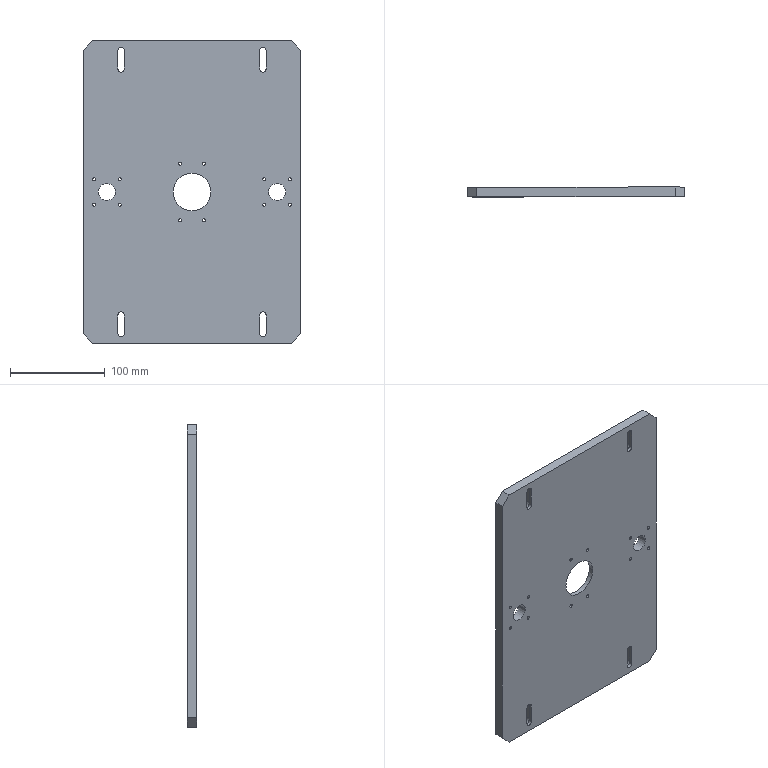Component | SolidWorks | UpperAndLowerCylinderMountingPlate-1 | 1 solid | 85 faces | box 230 x 10.04 x 320 mm | volume 691383 mm3 | cylinder 50 | plane 35 | commonest cylinder face diameters 3.3 x24 11 x8 6.6 x8 18 x4 8 x4 40 x2
build123d program:
from build123d import *

# Parameters (mm, degrees)
SKETCH1_W                                       = 230
SKETCH1_H                                       = 320
BOSS_EXTRUDE1_DEPTH                             = 10
SKETCH2_R                                       = 9
CUT_EXTRUDE1_DEPTH                              = 10
SKETCH3_R                                       = 20
CUT_EXTRUDE2_DEPTH                              = 10
CHAMFER1_SIZE                                   = 10
M4_TAPPED_HOLE1_D                               = 3.3
SKETCH6_W                                       = 50
SKETCH6_H                                       = 80
CUT_EXTRUDE3_DEPTH                              = 5
FILLET1_R                                       = 4
M4_TAPPED_HOLE2_D                               = 3.3
M6_HEX_SOCKET_HEAD_CAP_SCREW_CBORE1_D           = 6.6
M6_HEX_SOCKET_HEAD_CAP_SCREW_CBORE1_CBORE_D     = 11
M6_HEX_SOCKET_HEAD_CAP_SCREW_CBORE1_CBORE_DEPTH = 6.4
CUT_EXTRUDE4_DEPTH                              = 6.4
CUT_EXTRUDE5_DEPTH                              = 3.6


with BuildPart() as part:
    # Sketch1 → Boss-Extrude1 (new body)
    with BuildSketch(Plane.XY):
        Rectangle(SKETCH1_W, SKETCH1_H)
    extrude(amount=BOSS_EXTRUDE1_DEPTH)

    # Sketch2 → Cut-Extrude1 (cut)
    with BuildSketch(Plane.XY.offset(10)):
        with Locations((-90, 0)):
            Circle(SKETCH2_R)
        with Locations((90, 0)):
            Circle(SKETCH2_R)
    extrude(amount=-CUT_EXTRUDE1_DEPTH, mode=Mode.SUBTRACT)

    # Sketch3 → Cut-Extrude2 (cut)
    with BuildSketch(Plane.XY.offset(10)):
        Circle(SKETCH3_R)
    extrude(amount=-CUT_EXTRUDE2_DEPTH, mode=Mode.SUBTRACT)

    # Chamfer1
    chamfer1_edges = [part.edges().sort_by_distance(p)[0] for p in [
        (-115, 160, 5),
        (115, 160, 5),
        (115, -160, 5),
        (-115, -160, 5),
    ]]
    chamfer(chamfer1_edges, length=CHAMFER1_SIZE)

    # M4 Tapped Hole1 (through all)
    with Locations(Plane.XY.offset(10)):
        with Locations((-103.435, 13.435), (-76.565, 13.435), (-76.565, -13.435), (-103.435, -13.435)):
            m4_tapped_hole1 = Hole(M4_TAPPED_HOLE1_D / 2)

    # Mirror1: M4 Tapped Hole1 across plane
    add(m4_tapped_hole1.mirror(Plane(origin=(0, 0, 0), x_dir=(0, 0, 1), z_dir=(1, 0, 0))), mode=Mode.SUBTRACT)

    # Sketch6 → Cut-Extrude3 (cut)
    with BuildSketch(Plane.XY.offset(10)):
        Rectangle(SKETCH6_W, SKETCH6_H)
    extrude(amount=-CUT_EXTRUDE3_DEPTH, mode=Mode.SUBTRACT)

    # Fillet1
    fillet1_edges = [part.edges().sort_by_distance(p)[0] for p in [
        (-25, -40, 7.5),
        (-25, 40, 7.5),
        (25, 40, 7.5),
        (25, -40, 7.5),
    ]]
    fillet(fillet1_edges, radius=FILLET1_R)

    # M4 Tapped Hole2 (through all)
    with Locations(Plane.XY.offset(5)):
        with Locations((-12.5, 30), (12.5, 30), (-12.5, -30), (12.5, -30)):
            Hole(M4_TAPPED_HOLE2_D / 2)

    # M6 Hex Socket Head Cap Screw CBORE1 (through all)
    with Locations(Plane.XY.offset(10)):
        with Locations((-75, -140), (75, -140), (-75, 140), (75, 140)):
            CounterBoreHole(M6_HEX_SOCKET_HEAD_CAP_SCREW_CBORE1_D / 2, M6_HEX_SOCKET_HEAD_CAP_SCREW_CBORE1_CBORE_D / 2, M6_HEX_SOCKET_HEAD_CAP_SCREW_CBORE1_CBORE_DEPTH)

    # Sketch11 → Cut-Extrude4 (cut)
    with BuildSketch(Plane.XY.offset(10)):
        with BuildLine():
            Line((-69.5, 150), (-69.5, 130))
            ThreePointArc((-69.5, 130), (-75, 124.5), (-80.5, 130))
            Line((-80.5, 130), (-80.5, 150))
            ThreePointArc((-80.5, 150), (-75, 155.5), (-69.5, 150))
        make_face()
        with BuildLine():
            Line((80.5, 150), (80.5, 130))
            ThreePointArc((80.5, 130), (75, 124.5), (69.5, 130))
            Line((69.5, 130), (69.5, 150))
            ThreePointArc((69.5, 150), (75, 155.5), (80.5, 150))
        make_face()
        with BuildLine():
            Line((-69.5, -130), (-69.5, -150))
            ThreePointArc((-69.5, -150), (-75, -155.5), (-80.5, -150))
            Line((-80.5, -150), (-80.5, -130))
            ThreePointArc((-80.5, -130), (-75, -124.5), (-69.5, -130))
        make_face()
        with BuildLine():
            Line((80.5, -130), (80.5, -150))
            ThreePointArc((80.5, -150), (75, -155.5), (69.5, -150))
            Line((69.5, -150), (69.5, -130))
            ThreePointArc((69.5, -130), (75, -124.5), (80.5, -130))
        make_face()
    extrude(amount=-CUT_EXTRUDE4_DEPTH, mode=Mode.SUBTRACT)

    # Sketch12 → Cut-Extrude5 (cut)
    with BuildSketch(Plane.XY.offset(3.6)):
        with BuildLine():
            Line((-71.7, 150), (-71.7, 130))
            ThreePointArc((-71.7, 130), (-75, 126.7), (-78.3, 130))
            Line((-78.3, 130), (-78.3, 150))
            ThreePointArc((-78.3, 150), (-75, 153.3), (-71.7, 150))
        make_face()
        with BuildLine():
            Line((78.3, 150), (78.3, 130))
            ThreePointArc((78.3, 130), (75, 126.7), (71.7, 130))
            Line((71.7, 130), (71.7, 150))
            ThreePointArc((71.7, 150), (75, 153.3), (78.3, 150))
        make_face()
        with BuildLine():
            Line((78.3, -130), (78.3, -150))
            ThreePointArc((78.3, -150), (75, -153.3), (71.7, -150))
            Line((71.7, -150), (71.7, -130))
            ThreePointArc((71.7, -130), (75, -126.7), (78.3, -130))
        make_face()
        with BuildLine():
            Line((-71.7, -130), (-71.7, -150))
            ThreePointArc((-71.7, -150), (-75, -153.3), (-78.3, -150))
            Line((-78.3, -150), (-78.3, -130))
            ThreePointArc((-78.3, -130), (-75, -126.7), (-71.7, -130))
        make_face()
    extrude(amount=-CUT_EXTRUDE5_DEPTH, mode=Mode.SUBTRACT)


solid = part.part

# Placed as in the assembly
solid = solid.moved(Location((1702.143, 3963.72, 1079.241), (-90, -0.008895, 0)))